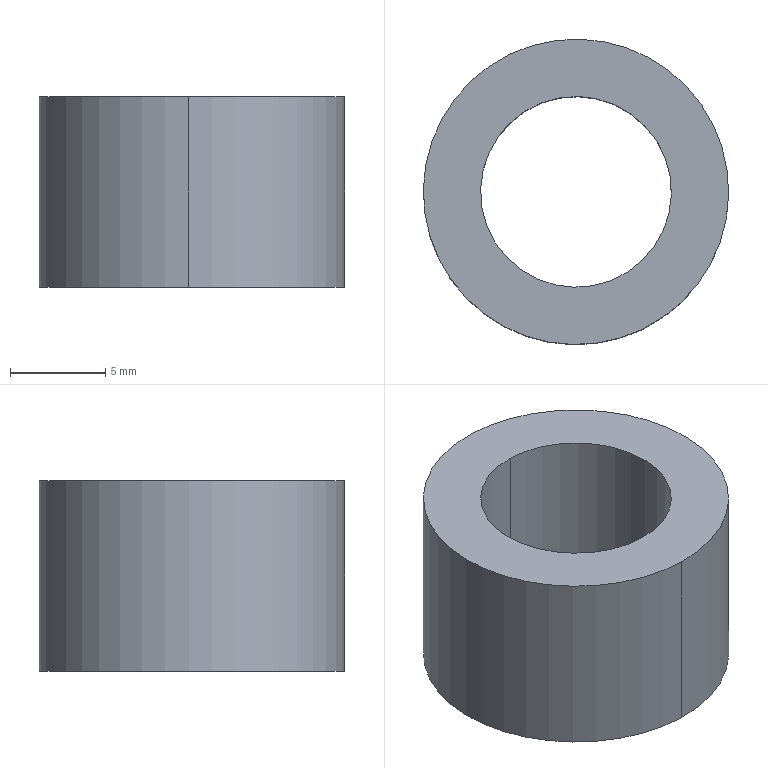Component | SolidWorks | Collar-2 | 1 solid | 6 faces | box 16 x 16 x 10 mm | volume 1225 mm3 | cylinder 4 | plane 2 | commonest cylinder face diameters 10 x2 16 x2
build123d program:
from build123d import *

# Parameters (mm, degrees)
SKETCH1_R           = 8
SKETCH1_R_2         = 5
BOSS_EXTRUDE1_DEPTH = 10


with BuildPart() as part:
    # Sketch1 → Boss-Extrude1 (new body)
    with BuildSketch(Plane(origin=(0, 0, 0), x_dir=(1, 0, 0), z_dir=(0, 1, 0))):
        with Locations(Location((0, 0, 0), (0, 0, 270))):
            Circle(SKETCH1_R)
        with Locations(Location((0, 0, 0), (0, 0, 270))):
            Circle(SKETCH1_R_2, mode=Mode.SUBTRACT)
    extrude(amount=BOSS_EXTRUDE1_DEPTH)


solid = part.part

# Placed as in the assembly
solid = solid.moved(Location((65.366, -4.894, 126.846), (90, 0, 0)))
STEP:
#1=COLOUR_RGB('',0.7922,0.8196,0.9333);
#2=FILL_AREA_STYLE_COLOUR('',#1);
#3=FILL_AREA_STYLE('',(#2));
#4=SURFACE_STYLE_FILL_AREA(#3);
#5=SURFACE_SIDE_STYLE('',(#4));
#6=SURFACE_STYLE_USAGE(.BOTH.,#5);
#7=PRESENTATION_STYLE_ASSIGNMENT((#6));
#8=CARTESIAN_POINT('',(2.578,0.004115,5.388));
#9=VERTEX_POINT('',#8);
#10=CARTESIAN_POINT('',(2.569,-0.3895,5.388));
#11=VERTEX_POINT('',#10);
#12=CARTESIAN_POINT('',(2.573,-0.1927,5.388));
#13=DIRECTION('',(0.,0.,1.));
#14=DIRECTION('',(-0.02278,-0.9997,0.));
#15=AXIS2_PLACEMENT_3D('',#12,#13,#14);
#16=CIRCLE('',#15,0.1969);
#17=EDGE_CURVE('',#9,#11,#16,.T.);
#18=ORIENTED_EDGE('',*,*,#17,.T.);
#19=CARTESIAN_POINT('',(2.569,-0.3895,4.994));
#20=VERTEX_POINT('',#19);
#21=CARTESIAN_POINT('',(2.569,-0.3895,5.388));
#22=DIRECTION('',(0.,0.,-1.));
#23=VECTOR('',#22,39.37);
#24=LINE('',#21,#23);
#25=EDGE_CURVE('',#11,#20,#24,.T.);
#26=ORIENTED_EDGE('',*,*,#25,.T.);
#27=CARTESIAN_POINT('',(2.578,0.004115,4.994));
#28=VERTEX_POINT('',#27);
#29=CARTESIAN_POINT('',(2.573,-0.1927,4.994));
#30=DIRECTION('',(0.,0.,1.));
#31=DIRECTION('',(-0.02278,-0.9997,0.));
#32=AXIS2_PLACEMENT_3D('',#29,#30,#31);
#33=CIRCLE('',#32,0.1969);
#34=EDGE_CURVE('',#28,#20,#33,.T.);
#35=ORIENTED_EDGE('',*,*,#34,.F.);
#36=CARTESIAN_POINT('',(2.578,0.004115,5.388));
#37=DIRECTION('',(0.,0.,-1.));
#38=VECTOR('',#37,39.37);
#39=LINE('',#36,#38);
#40=EDGE_CURVE('',#9,#28,#39,.T.);
#41=ORIENTED_EDGE('',*,*,#40,.F.);
#42=EDGE_LOOP('',(#18,#26,#35,#41));
#43=FACE_OUTER_BOUND('',#42,.T.);
#44=CARTESIAN_POINT('',(2.573,-0.1927,5.388));
#45=DIRECTION('',(0.,0.,-1.));
#46=DIRECTION('',(0.02278,0.9997,0.));
#47=AXIS2_PLACEMENT_3D('',#44,#45,#46);
#48=CYLINDRICAL_SURFACE('',#47,0.1969);
#49=ADVANCED_FACE('',(#43),#48,.F.);
#50=CARTESIAN_POINT('',(2.566,-0.5076,5.388));
#51=VERTEX_POINT('',#50);
#52=CARTESIAN_POINT('',(2.581,0.1222,5.388));
#53=VERTEX_POINT('',#52);
#54=CARTESIAN_POINT('',(2.573,-0.1927,5.388));
#55=DIRECTION('',(0.,0.,1.));
#56=DIRECTION('',(-0.02278,-0.9997,0.));
#57=AXIS2_PLACEMENT_3D('',#54,#55,#56);
#58=CIRCLE('',#57,0.315);
#59=EDGE_CURVE('',#51,#53,#58,.T.);
#60=ORIENTED_EDGE('',*,*,#59,.F.);
#61=CARTESIAN_POINT('',(2.566,-0.5076,4.994));
#62=VERTEX_POINT('',#61);
#63=CARTESIAN_POINT('',(2.566,-0.5076,5.388));
#64=DIRECTION('',(0.,0.,-1.));
#65=VECTOR('',#64,39.37);
#66=LINE('',#63,#65);
#67=EDGE_CURVE('',#51,#62,#66,.T.);
#68=ORIENTED_EDGE('',*,*,#67,.T.);
#69=CARTESIAN_POINT('',(2.581,0.1222,4.994));
#70=VERTEX_POINT('',#69);
#71=CARTESIAN_POINT('',(2.573,-0.1927,4.994));
#72=DIRECTION('',(0.,0.,1.));
#73=DIRECTION('',(-0.02278,-0.9997,0.));
#74=AXIS2_PLACEMENT_3D('',#71,#72,#73);
#75=CIRCLE('',#74,0.315);
#76=EDGE_CURVE('',#62,#70,#75,.T.);
#77=ORIENTED_EDGE('',*,*,#76,.T.);
#78=CARTESIAN_POINT('',(2.581,0.1222,5.388));
#79=DIRECTION('',(0.,0.,-1.));
#80=VECTOR('',#79,39.37);
#81=LINE('',#78,#80);
#82=EDGE_CURVE('',#53,#70,#81,.T.);
#83=ORIENTED_EDGE('',*,*,#82,.F.);
#84=EDGE_LOOP('',(#60,#68,#77,#83));
#85=FACE_OUTER_BOUND('',#84,.T.);
#86=CARTESIAN_POINT('',(2.573,-0.1927,5.388));
#87=DIRECTION('',(0.,0.,-1.));
#88=DIRECTION('',(0.02278,0.9997,0.));
#89=AXIS2_PLACEMENT_3D('',#86,#87,#88);
#90=CYLINDRICAL_SURFACE('',#89,0.315);
#91=ADVANCED_FACE('',(#85),#90,.T.);
#92=CARTESIAN_POINT('',(2.573,-0.1927,5.388));
#93=DIRECTION('',(0.,0.,1.));
#94=DIRECTION('',(-0.02278,-0.9997,0.));
#95=AXIS2_PLACEMENT_3D('',#92,#93,#94);
#96=CIRCLE('',#95,0.315);
#97=EDGE_CURVE('',#53,#51,#96,.T.);
#98=ORIENTED_EDGE('',*,*,#97,.T.);
#99=ORIENTED_EDGE('',*,*,#59,.T.);
#100=EDGE_LOOP('',(#98,#99));
#101=FACE_OUTER_BOUND('',#100,.T.);
#102=ORIENTED_EDGE('',*,*,#17,.F.);
#103=CARTESIAN_POINT('',(2.573,-0.1927,5.388));
#104=DIRECTION('',(0.,0.,1.));
#105=DIRECTION('',(-0.02278,-0.9997,0.));
#106=AXIS2_PLACEMENT_3D('',#103,#104,#105);
#107=CIRCLE('',#106,0.1969);
#108=EDGE_CURVE('',#11,#9,#107,.T.);
#109=ORIENTED_EDGE('',*,*,#108,.F.);
#110=EDGE_LOOP('',(#102,#109));
#111=FACE_BOUND('',#110,.T.);
#112=CARTESIAN_POINT('',(2.573,-0.1927,5.388));
#113=DIRECTION('',(0.,0.,1.));
#114=DIRECTION('',(-0.02278,-0.9997,0.));
#115=AXIS2_PLACEMENT_3D('',#112,#113,#114);
#116=PLANE('',#115);
#117=ADVANCED_FACE('',(#101,#111),#116,.T.);
#118=CARTESIAN_POINT('',(2.573,-0.1927,4.994));
#119=DIRECTION('',(0.,0.,1.));
#120=DIRECTION('',(-0.02278,-0.9997,0.));
#121=AXIS2_PLACEMENT_3D('',#118,#119,#120);
#122=CIRCLE('',#121,0.315);
#123=EDGE_CURVE('',#70,#62,#122,.T.);
#124=ORIENTED_EDGE('',*,*,#123,.F.);
#125=ORIENTED_EDGE('',*,*,#76,.F.);
#126=EDGE_LOOP('',(#124,#125));
#127=FACE_OUTER_BOUND('',#126,.T.);
#128=ORIENTED_EDGE('',*,*,#34,.T.);
#129=CARTESIAN_POINT('',(2.573,-0.1927,4.994));
#130=DIRECTION('',(0.,0.,1.));
#131=DIRECTION('',(-0.02278,-0.9997,0.));
#132=AXIS2_PLACEMENT_3D('',#129,#130,#131);
#133=CIRCLE('',#132,0.1969);
#134=EDGE_CURVE('',#20,#28,#133,.T.);
#135=ORIENTED_EDGE('',*,*,#134,.T.);
#136=EDGE_LOOP('',(#128,#135));
#137=FACE_BOUND('',#136,.T.);
#138=CARTESIAN_POINT('',(2.573,-0.1927,4.994));
#139=DIRECTION('',(0.,0.,1.));
#140=DIRECTION('',(-0.02278,-0.9997,0.));
#141=AXIS2_PLACEMENT_3D('',#138,#139,#140);
#142=PLANE('',#141);
#143=ADVANCED_FACE('',(#127,#137),#142,.F.);
#144=ORIENTED_EDGE('',*,*,#67,.F.);
#145=ORIENTED_EDGE('',*,*,#97,.F.);
#146=ORIENTED_EDGE('',*,*,#82,.T.);
#147=ORIENTED_EDGE('',*,*,#123,.T.);
#148=EDGE_LOOP('',(#144,#145,#146,#147));
#149=FACE_OUTER_BOUND('',#148,.T.);
#150=CARTESIAN_POINT('',(2.573,-0.1927,5.388));
#151=DIRECTION('',(0.,0.,-1.));
#152=DIRECTION('',(0.02278,0.9997,0.));
#153=AXIS2_PLACEMENT_3D('',#150,#151,#152);
#154=CYLINDRICAL_SURFACE('',#153,0.315);
#155=ADVANCED_FACE('',(#149),#154,.T.);
#156=ORIENTED_EDGE('',*,*,#25,.F.);
#157=ORIENTED_EDGE('',*,*,#108,.T.);
#158=ORIENTED_EDGE('',*,*,#40,.T.);
#159=ORIENTED_EDGE('',*,*,#134,.F.);
#160=EDGE_LOOP('',(#156,#157,#158,#159));
#161=FACE_OUTER_BOUND('',#160,.T.);
#162=CARTESIAN_POINT('',(2.573,-0.1927,5.388));
#163=DIRECTION('',(0.,0.,-1.));
#164=DIRECTION('',(0.02278,0.9997,0.));
#165=AXIS2_PLACEMENT_3D('',#162,#163,#164);
#166=CYLINDRICAL_SURFACE('',#165,0.1969);
#167=ADVANCED_FACE('',(#161),#166,.F.);
#168=CLOSED_SHELL('',(#49,#91,#117,#143,#155,#167));
#169=MANIFOLD_SOLID_BREP('',#168);
#170=STYLED_ITEM('',(#7),#169);
#171=(LENGTH_UNIT()NAMED_UNIT(*)SI_UNIT($,.METRE.));
#172=LENGTH_MEASURE_WITH_UNIT(LENGTH_MEASURE(0.0254),#171);
#173=DIMENSIONAL_EXPONENTS(1.,0.,0.,0.,0.,0.,0.);
#174=(CONVERSION_BASED_UNIT('',#172)LENGTH_UNIT()NAMED_UNIT(#173));
#175=UNCERTAINTY_MEASURE_WITH_UNIT(LENGTH_MEASURE(0.00001),#174,'','');
#176=(NAMED_UNIT(*)PLANE_ANGLE_UNIT()SI_UNIT($,.RADIAN.));
#177=(NAMED_UNIT(*)SI_UNIT($,.STERADIAN.)SOLID_ANGLE_UNIT());
#178=(GEOMETRIC_REPRESENTATION_CONTEXT(3)GLOBAL_UNCERTAINTY_ASSIGNED_CONTEXT((#175))GLOBAL_UNIT_ASSIGNED_CONTEXT((#174,#176,#177))REPRESENTATION_CONTEXT('',''));
#179=MECHANICAL_DESIGN_GEOMETRIC_PRESENTATION_REPRESENTATION('',(#170),#178);
#180=PRESENTATION_LAYER_ASSIGNMENT('','',(#170));
#181=CARTESIAN_POINT('',(0.,0.,0.));
#182=DIRECTION('',(0.,0.,1.));
#183=DIRECTION('',(1.,0.,0.));
#184=AXIS2_PLACEMENT_3D('',#181,#182,#183);
#185=(LENGTH_UNIT()NAMED_UNIT(*)SI_UNIT($,.METRE.));
#186=LENGTH_MEASURE_WITH_UNIT(LENGTH_MEASURE(0.0254),#185);
#187=DIMENSIONAL_EXPONENTS(1.,0.,0.,0.,0.,0.,0.);
#188=(CONVERSION_BASED_UNIT('',#186)LENGTH_UNIT()NAMED_UNIT(#187));
#189=UNCERTAINTY_MEASURE_WITH_UNIT(LENGTH_MEASURE(0.00001),#188,'','');
#190=(NAMED_UNIT(*)PLANE_ANGLE_UNIT()SI_UNIT($,.RADIAN.));
#191=(NAMED_UNIT(*)SI_UNIT($,.STERADIAN.)SOLID_ANGLE_UNIT());
#192=(GEOMETRIC_REPRESENTATION_CONTEXT(3)GLOBAL_UNCERTAINTY_ASSIGNED_CONTEXT((#189))GLOBAL_UNIT_ASSIGNED_CONTEXT((#188,#190,#191))REPRESENTATION_CONTEXT('',''));
#193=ADVANCED_BREP_SHAPE_REPRESENTATION('',(#169,#184),#192);